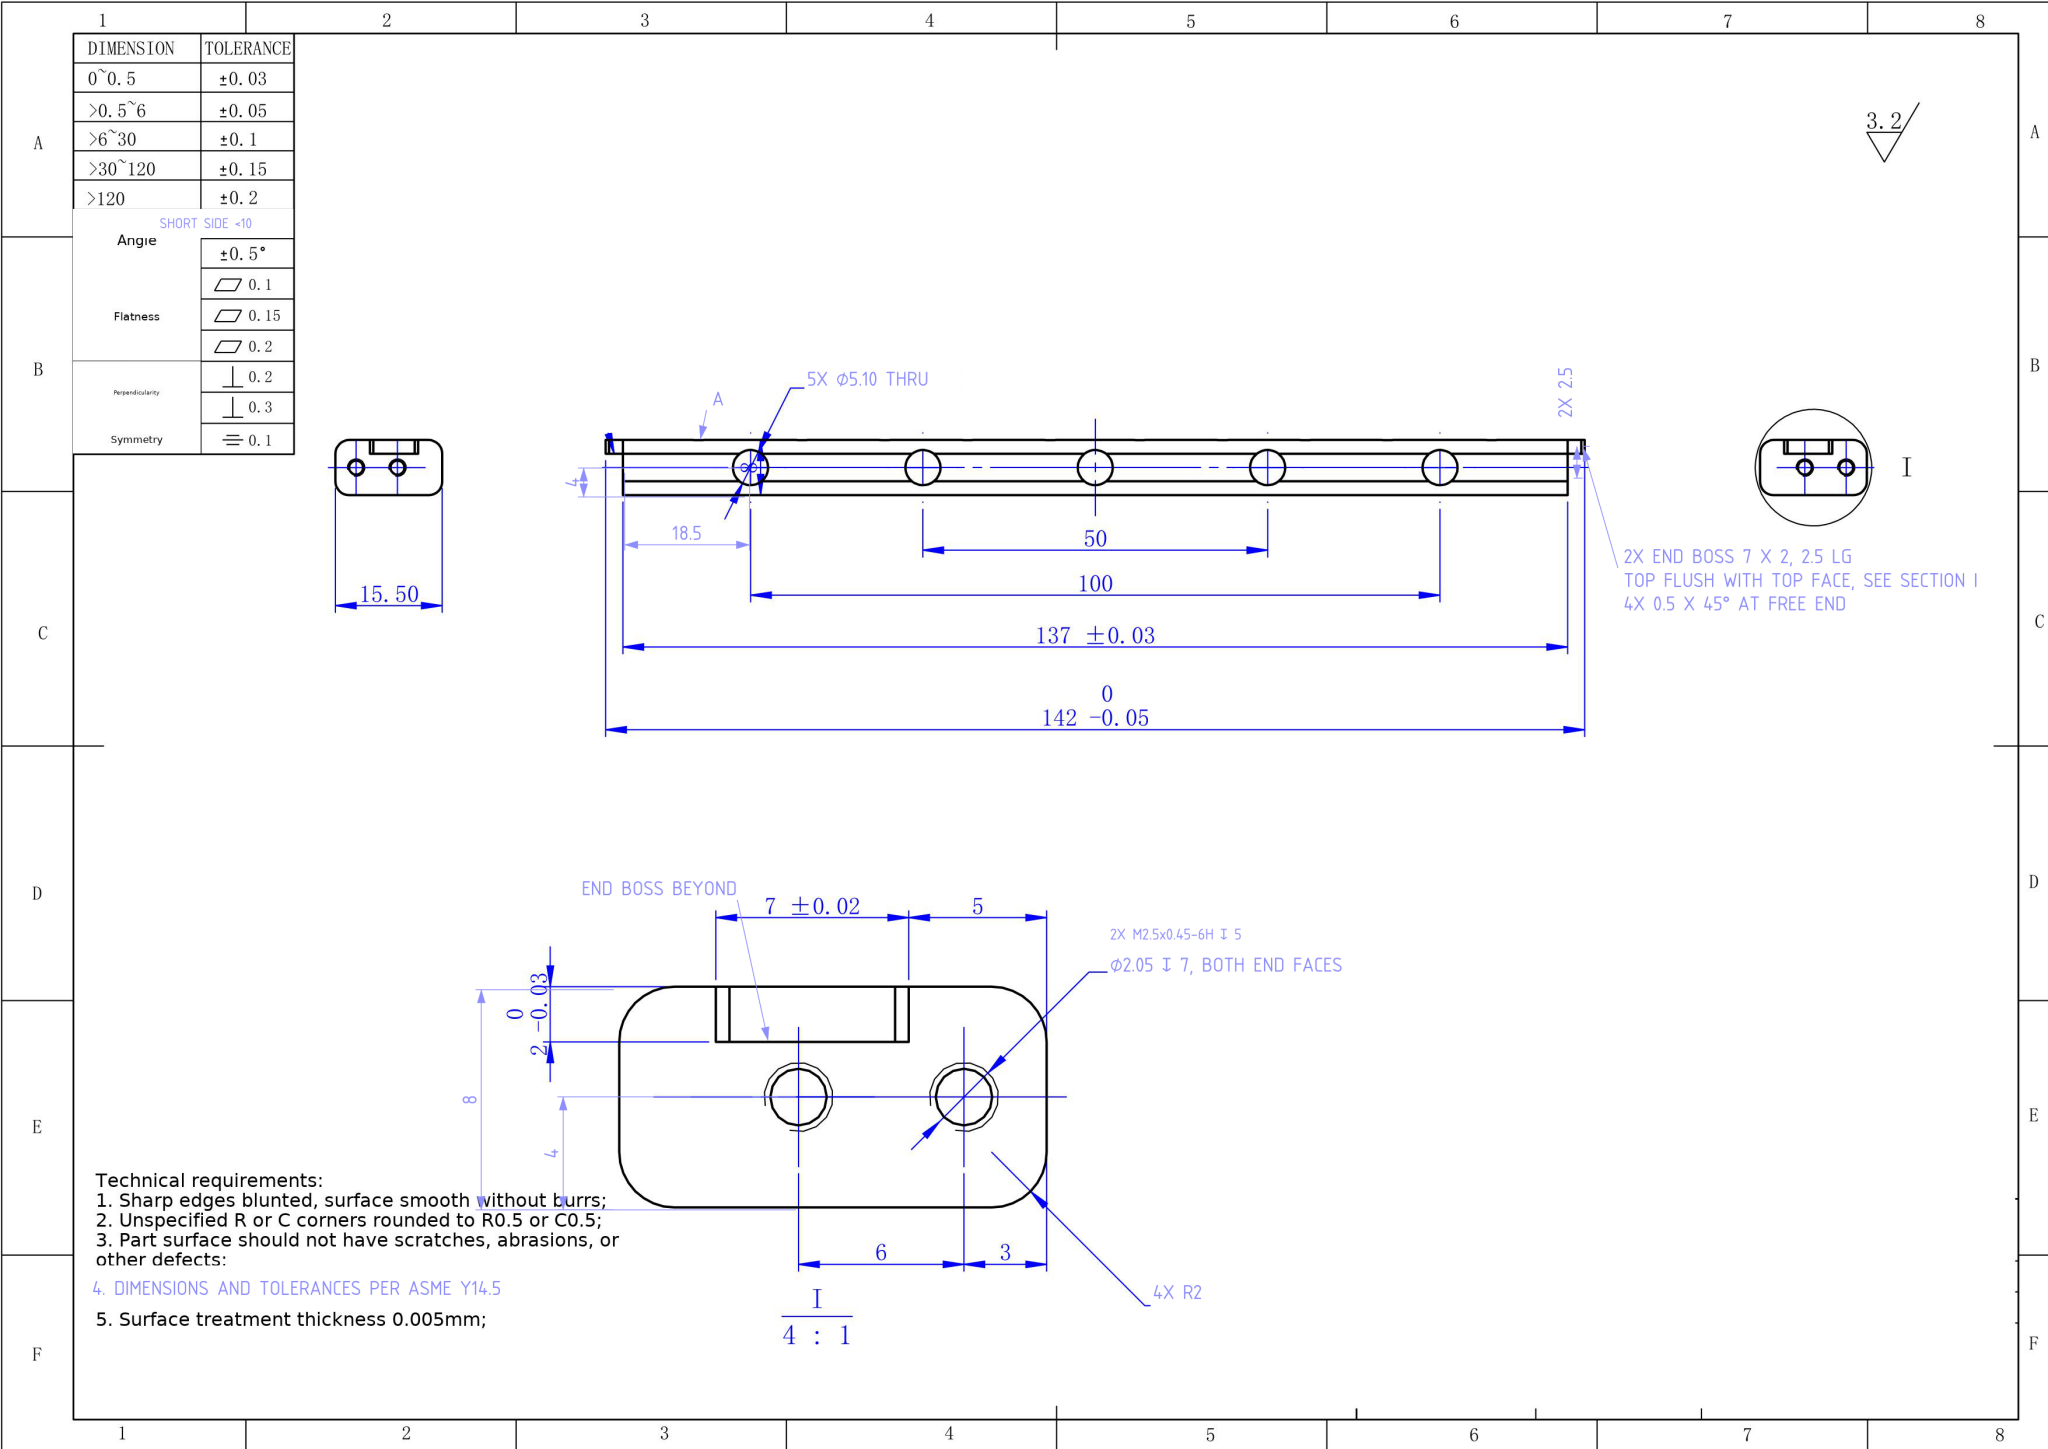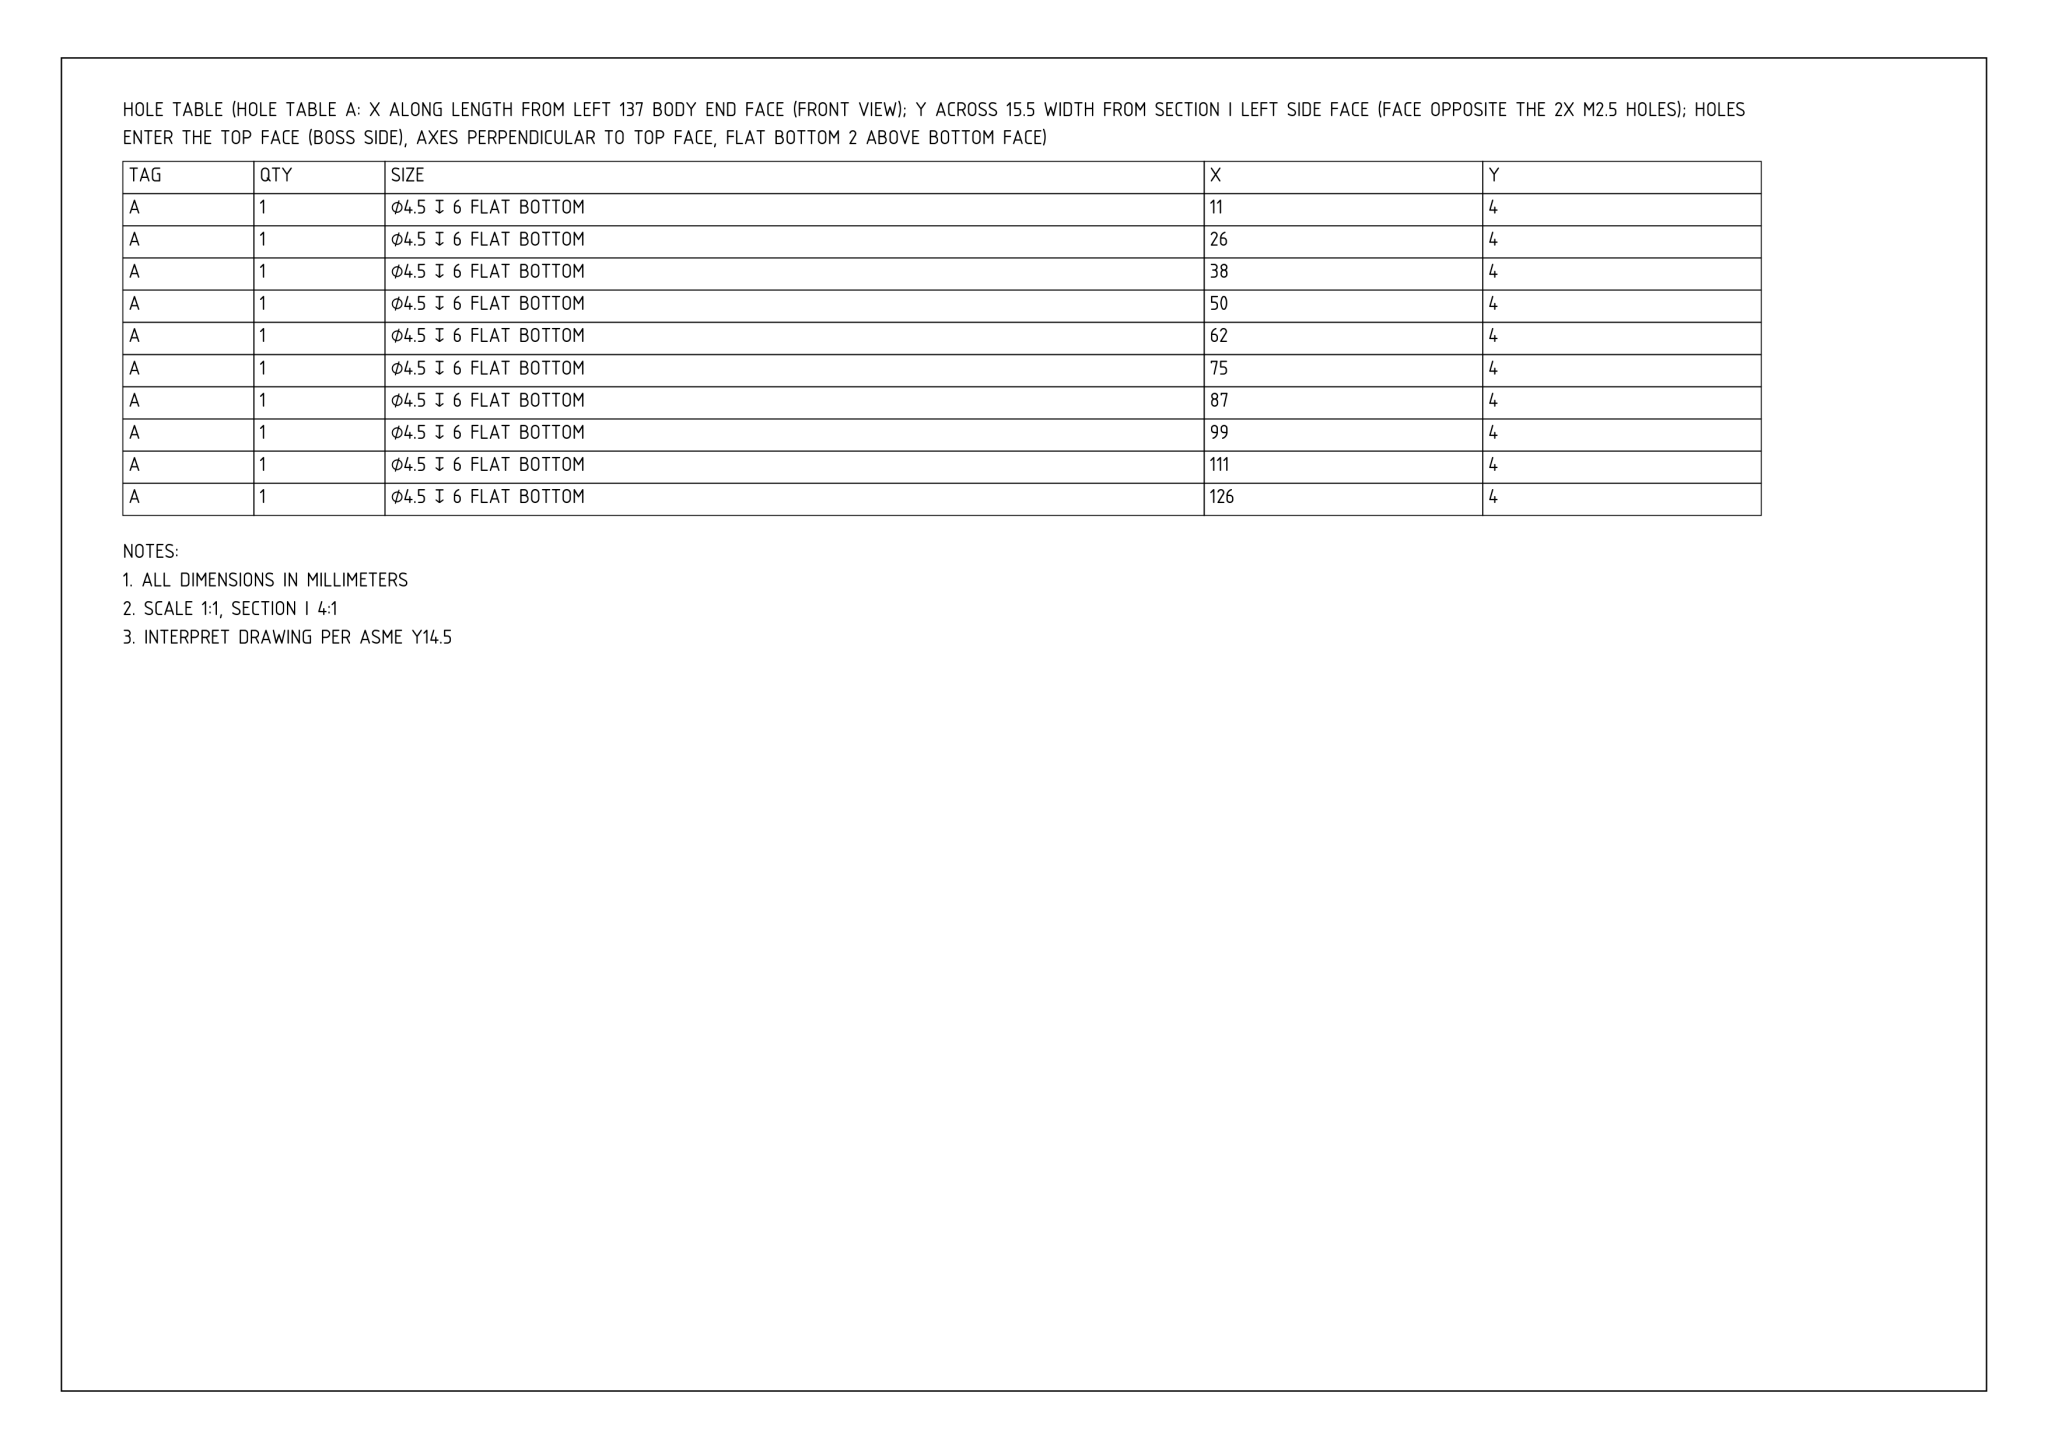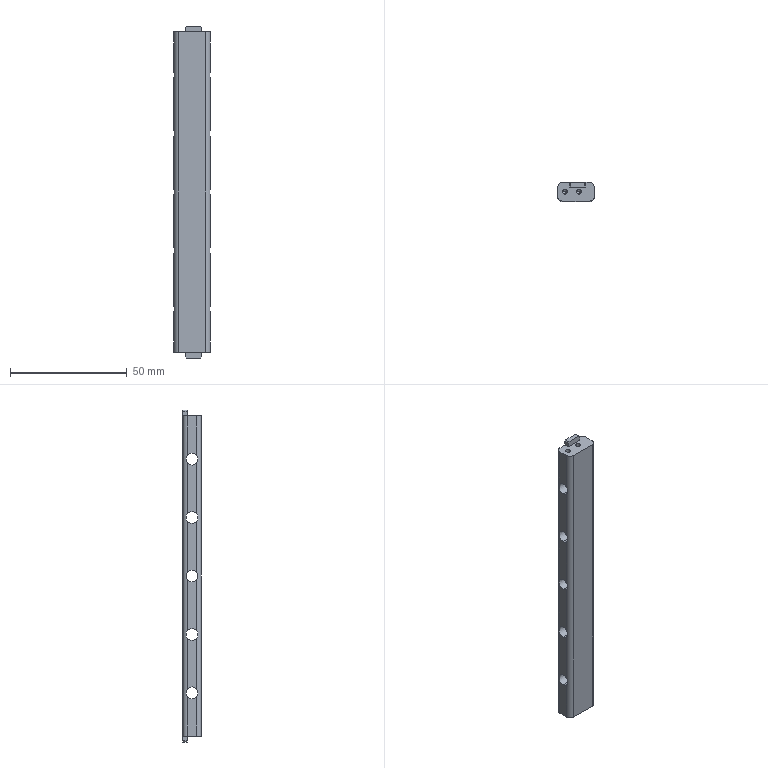Part | NX | mm | 1 solid | 88 faces | box 15.5 x 8 x 142 mm | volume 13946 mm3 | cylinder 42 | plane 38 | cone 8 | commonest cylinder face diameters 4.5 x20 5.1 x10 2.05 x8 4 x4